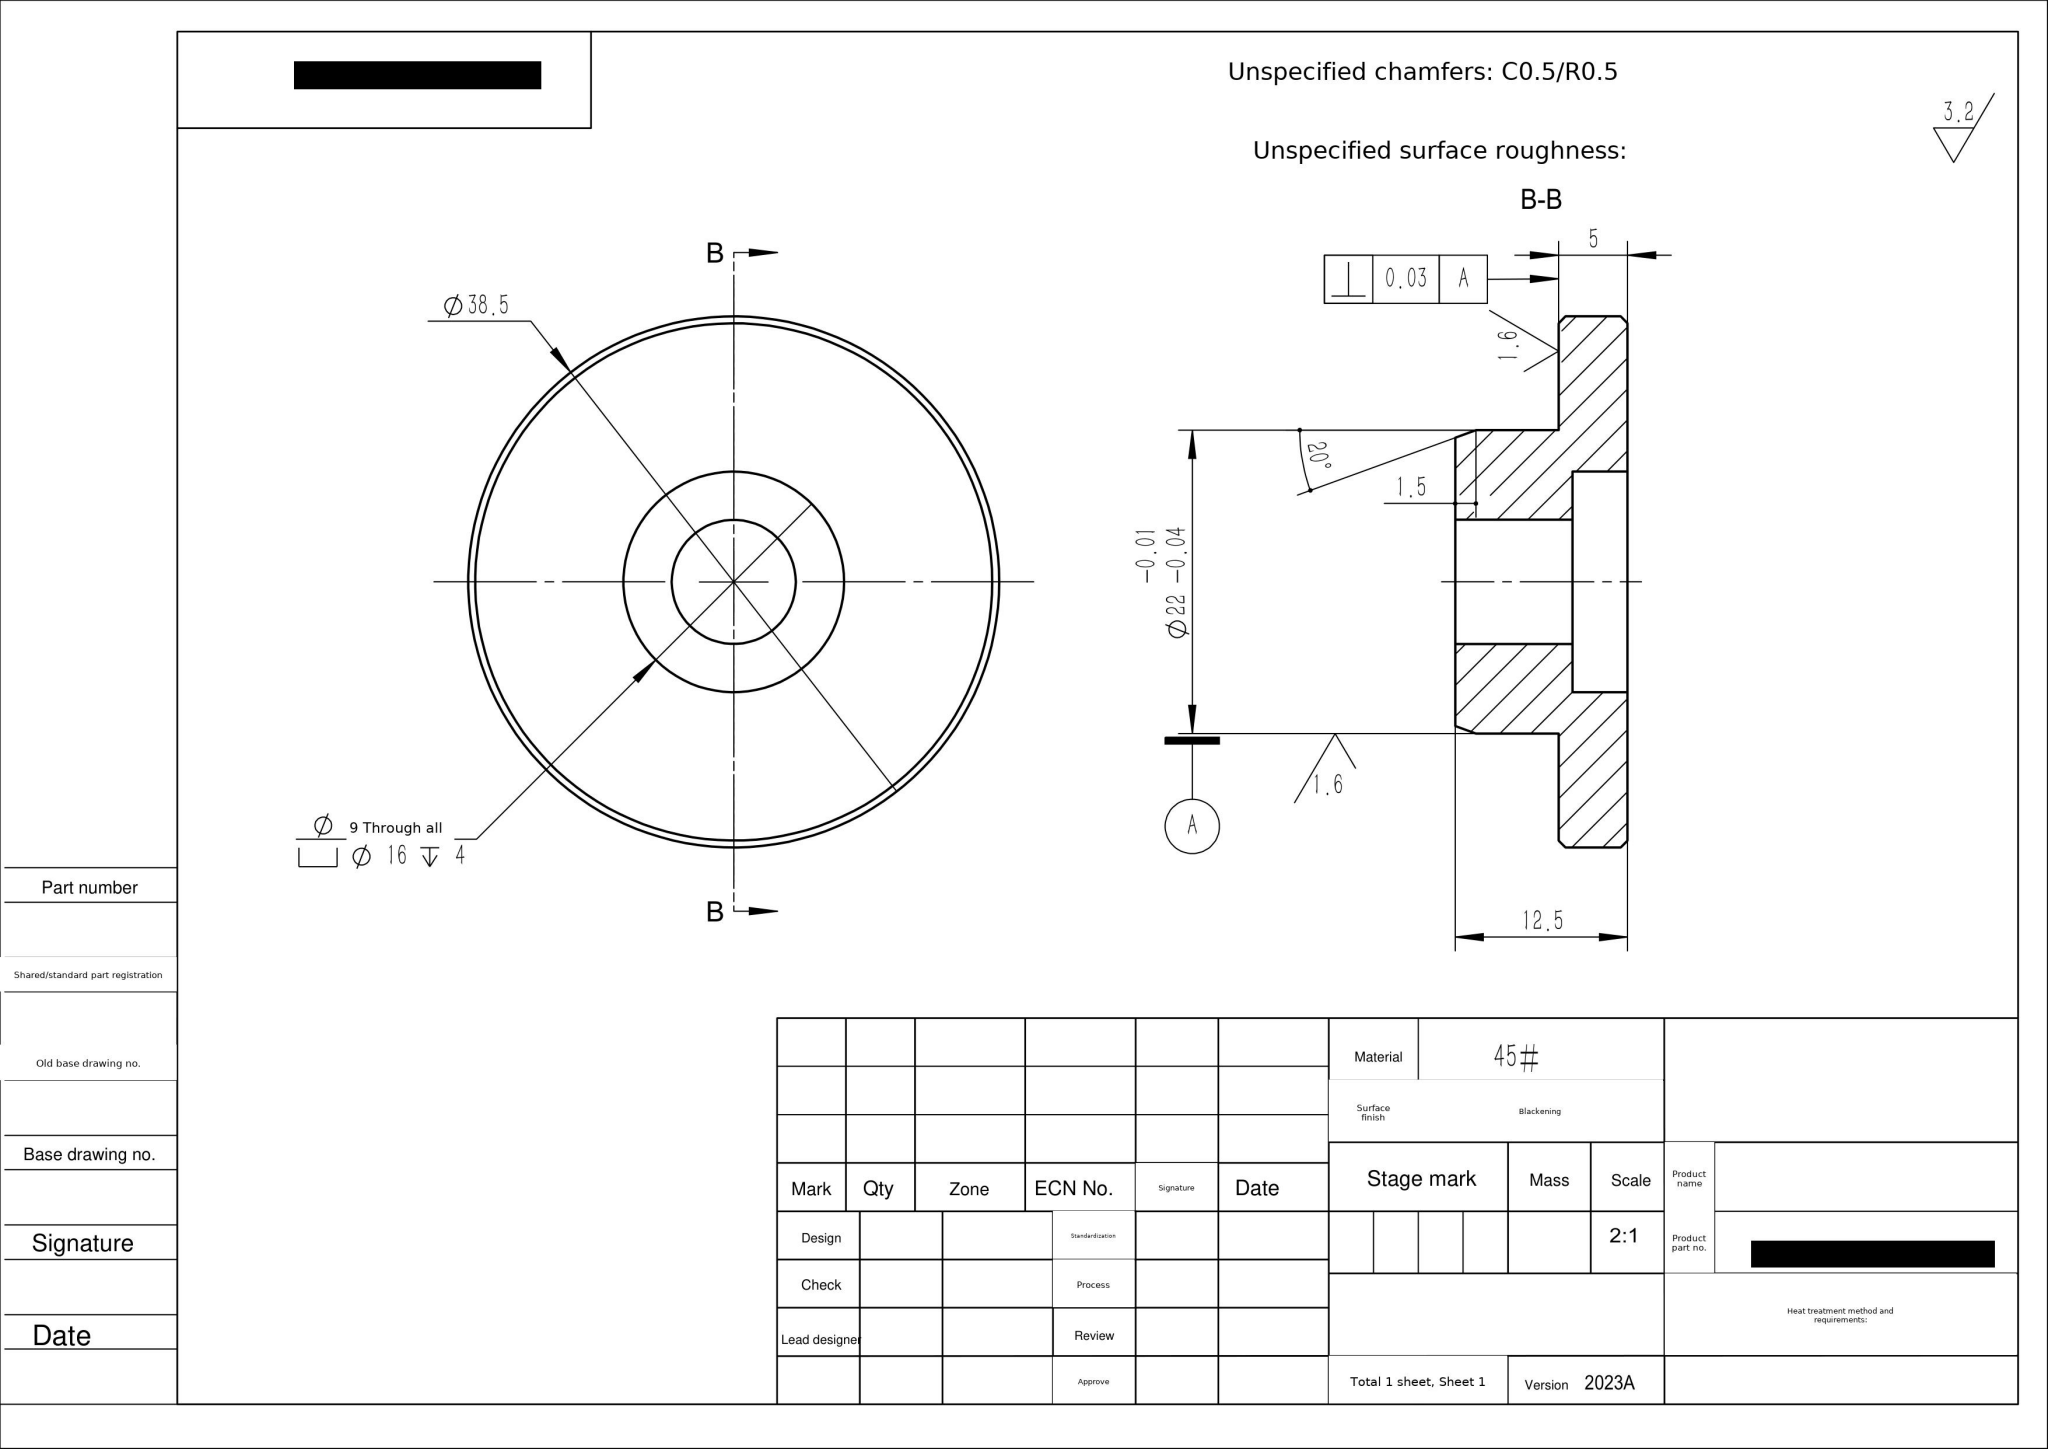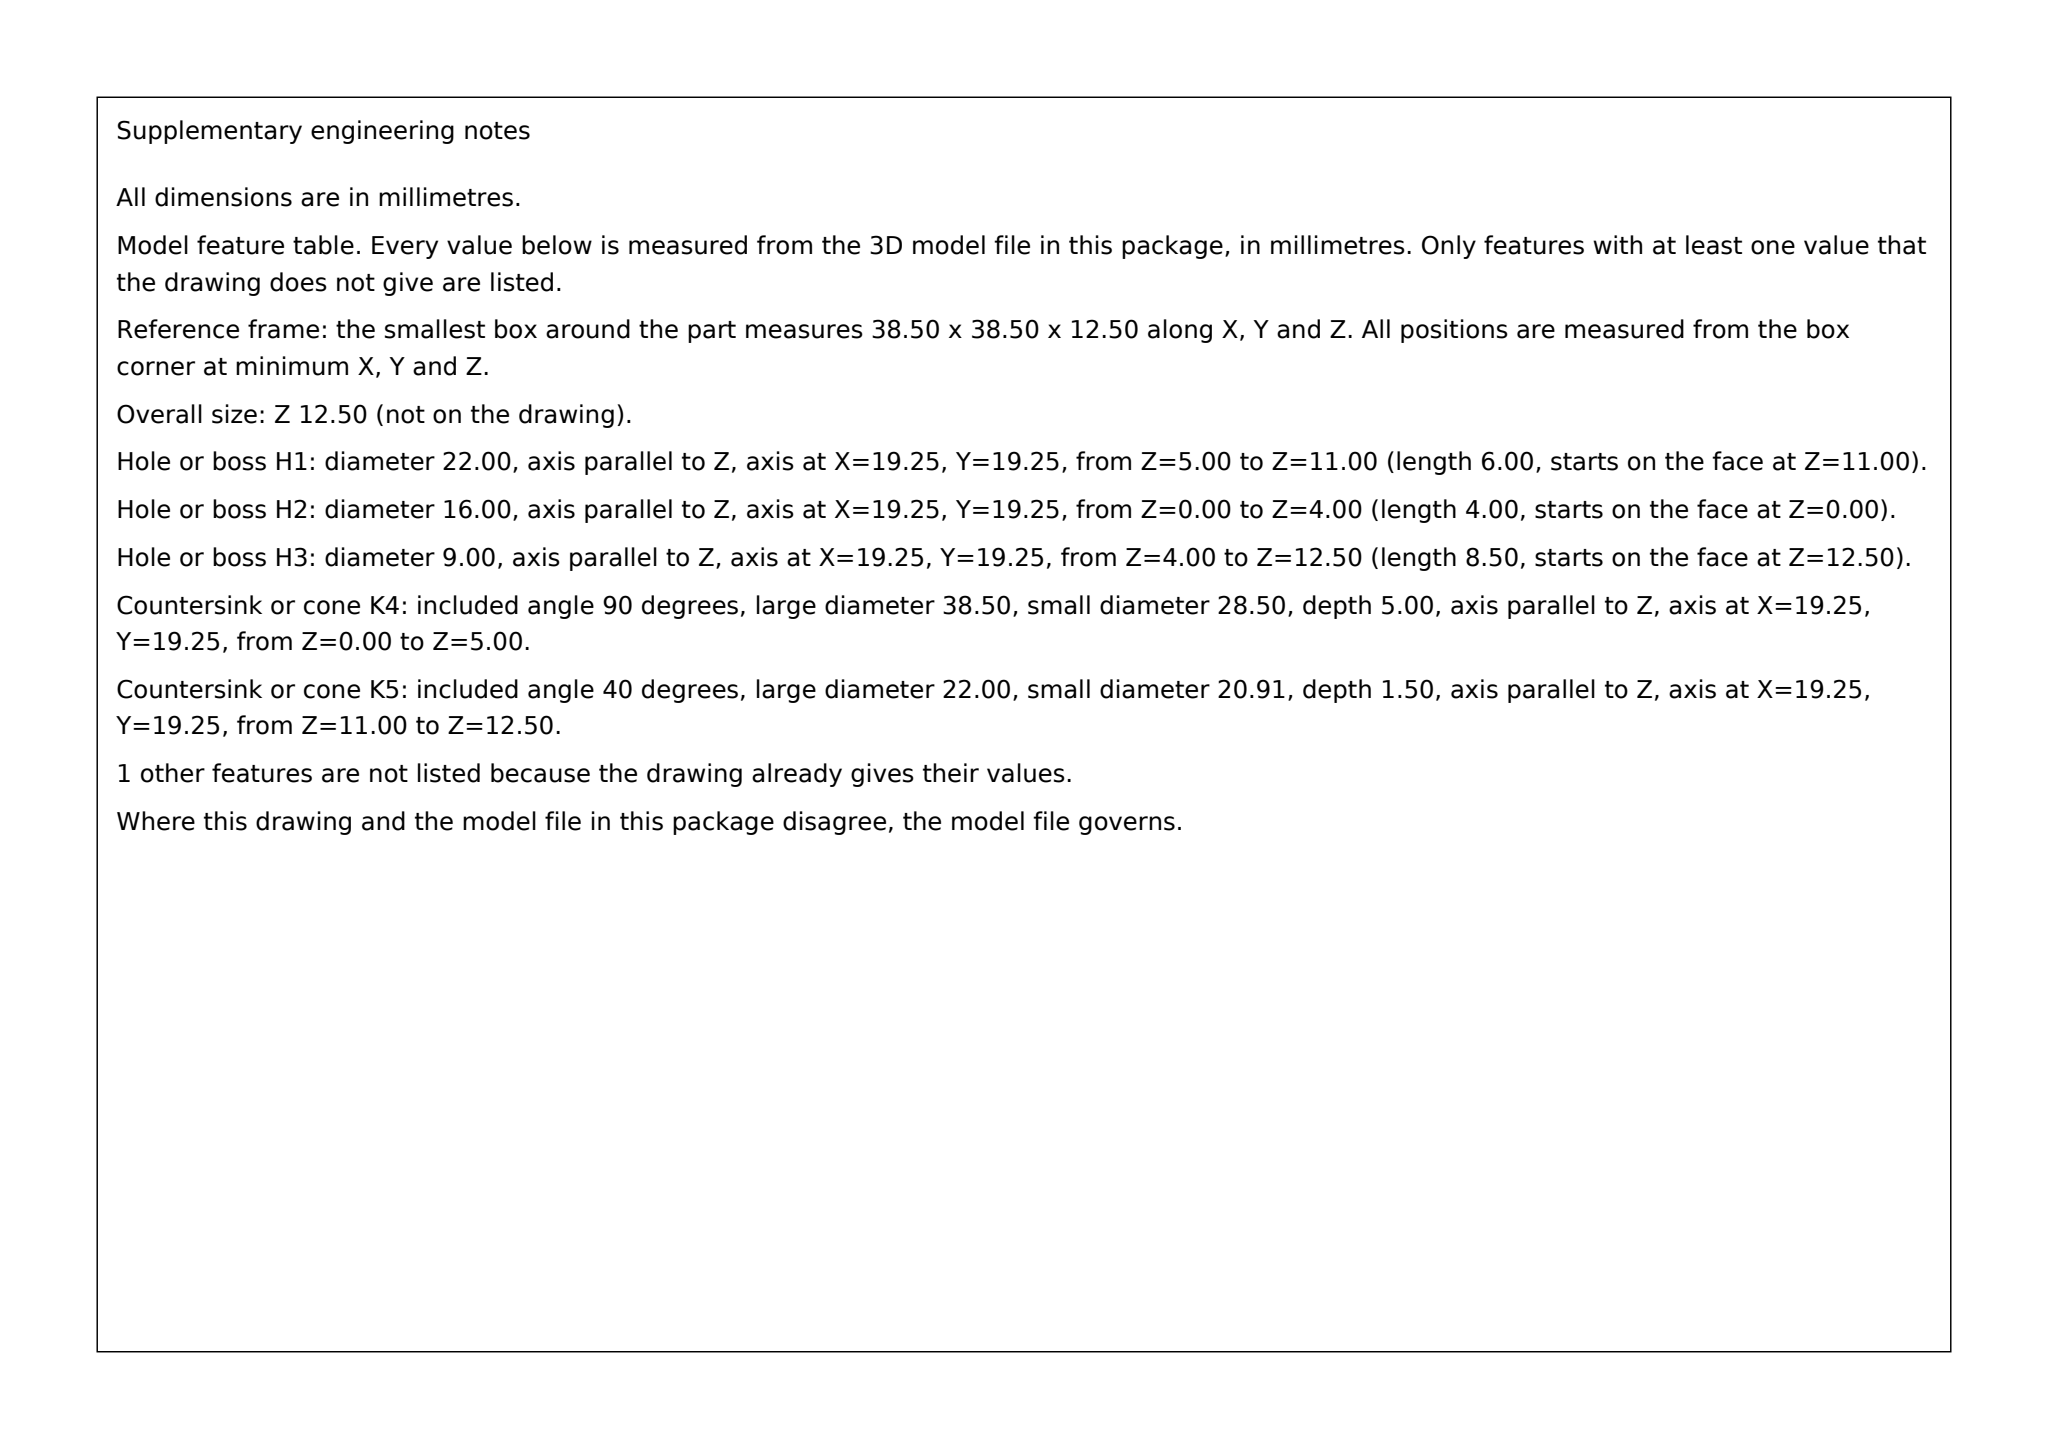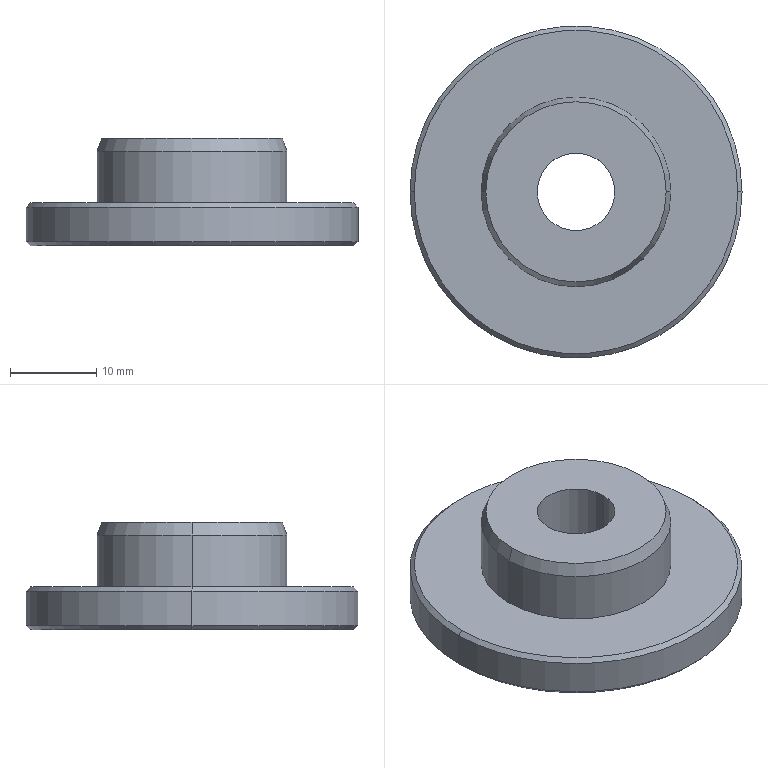Part | SolidWorks | mm | material 45# | 1 solid | 18 faces | box 38.5 x 38.5 x 12.5 mm | volume 7269 mm3 | cylinder 8 | cone 6 | plane 4 | commonest cylinder face diameters 16 x2 9 x2 38.5 x2 22 x2
build123d program:
from build123d import *

# Parameters (mm, degrees)
SKETCH1_R                                            = 11
BOSS_EXTRUDE1_DEPTH                                  = 7.5
SKETCH2_R                                            = 19.25
BOSS_EXTRUDE2_DEPTH                                  = 5
CHAMFER1_SIZE                                        = 1.5
CHAMFER1_SIZE2                                       = 0.546
CHAMFER2_SIZE                                        = 0.5
HOLE_SIZE_ACCORDING_TO_TYPE_1_OF_HEXAGON_D           = 9
HOLE_SIZE_ACCORDING_TO_TYPE_1_OF_HEXAGON_CBORE_D     = 16
HOLE_SIZE_ACCORDING_TO_TYPE_1_OF_HEXAGON_CBORE_DEPTH = 4


with BuildPart() as part:
    # Sketch1 → Boss-Extrude1 (new body)
    with BuildSketch(Plane.XY):
        Circle(SKETCH1_R)
    extrude(amount=BOSS_EXTRUDE1_DEPTH)

    # Sketch2 → Boss-Extrude2 (add)
    with BuildSketch(Plane(origin=(0, 0, 0), x_dir=(-1, 0, 0), z_dir=(0, 0, -1))):
        Circle(SKETCH2_R)
    extrude(amount=BOSS_EXTRUDE2_DEPTH)

    # Chamfer1
    chamfer1_edges = [part.edges().sort_by_distance(p)[0] for p in [
        (-11, 0, 7.5),
    ]]
    chamfer1_side = [part.faces().sort_by_distance(p)[0] for p in [
        (-11, 0, 3.75),
    ]]
    chamfer(chamfer1_edges, length=CHAMFER1_SIZE, length2=CHAMFER1_SIZE2, reference=chamfer1_side[0])

    # Chamfer2
    chamfer2_edges = [part.edges().sort_by_distance(p)[0] for p in [
        (19.25, 0, 0),
        (19.25, 0, -5),
    ]]
    chamfer(chamfer2_edges, length=CHAMFER2_SIZE)

    # Hole Size_According to_Type 1 of Hexagon (through all)
    with Locations(Plane(origin=(0, 0, -5), x_dir=(-1, 0, 0), z_dir=(0, 0, -1))):
        with Locations((0, 0)):
            CounterBoreHole(HOLE_SIZE_ACCORDING_TO_TYPE_1_OF_HEXAGON_D / 2, HOLE_SIZE_ACCORDING_TO_TYPE_1_OF_HEXAGON_CBORE_D / 2, HOLE_SIZE_ACCORDING_TO_TYPE_1_OF_HEXAGON_CBORE_DEPTH)


solid = part.part
STEP:
#1=CARTESIAN_POINT('',(8.,0.,-1.));
#2=VERTEX_POINT('',#1);
#3=CARTESIAN_POINT('',(-8.,0.,-1.));
#4=VERTEX_POINT('',#3);
#5=CARTESIAN_POINT('',(0.,0.,-1.));
#6=DIRECTION('',(0.,0.,-1.));
#7=DIRECTION('',(-1.,0.,0.));
#8=AXIS2_PLACEMENT_3D('',#5,#6,#7);
#9=CIRCLE('',#8,8.);
#10=EDGE_CURVE('',#2,#4,#9,.T.);
#11=ORIENTED_EDGE('',*,*,#10,.F.);
#12=CARTESIAN_POINT('',(8.,0.,-5.));
#13=VERTEX_POINT('',#12);
#14=CARTESIAN_POINT('',(8.,0.,-5.));
#15=DIRECTION('',(0.,0.,-1.));
#16=VECTOR('',#15,1000.);
#17=LINE('',#14,#16);
#18=EDGE_CURVE('',#2,#13,#17,.T.);
#19=ORIENTED_EDGE('',*,*,#18,.T.);
#20=CARTESIAN_POINT('',(-8.,0.,-5.));
#21=VERTEX_POINT('',#20);
#22=CARTESIAN_POINT('',(0.,0.,-5.));
#23=DIRECTION('',(0.,0.,-1.));
#24=DIRECTION('',(-1.,0.,0.));
#25=AXIS2_PLACEMENT_3D('',#22,#23,#24);
#26=CIRCLE('',#25,8.);
#27=EDGE_CURVE('',#13,#21,#26,.T.);
#28=ORIENTED_EDGE('',*,*,#27,.T.);
#29=CARTESIAN_POINT('',(-8.,0.,-5.));
#30=DIRECTION('',(0.,0.,-1.));
#31=VECTOR('',#30,1000.);
#32=LINE('',#29,#31);
#33=EDGE_CURVE('',#4,#21,#32,.T.);
#34=ORIENTED_EDGE('',*,*,#33,.F.);
#35=EDGE_LOOP('',(#11,#19,#28,#34));
#36=FACE_OUTER_BOUND('',#35,.T.);
#37=CARTESIAN_POINT('',(0.,0.,-5.));
#38=DIRECTION('',(0.,0.,-1.));
#39=DIRECTION('',(-1.,0.,0.));
#40=AXIS2_PLACEMENT_3D('',#37,#38,#39);
#41=CYLINDRICAL_SURFACE('',#40,8.);
#42=ADVANCED_FACE('',(#36),#41,.F.);
#43=CARTESIAN_POINT('',(4.5,0.,7.5));
#44=VERTEX_POINT('',#43);
#45=CARTESIAN_POINT('',(-4.5,0.,7.5));
#46=VERTEX_POINT('',#45);
#47=CARTESIAN_POINT('',(0.,0.,7.5));
#48=DIRECTION('',(0.,0.,-1.));
#49=DIRECTION('',(-1.,0.,0.));
#50=AXIS2_PLACEMENT_3D('',#47,#48,#49);
#51=CIRCLE('',#50,4.5);
#52=EDGE_CURVE('',#44,#46,#51,.T.);
#53=ORIENTED_EDGE('',*,*,#52,.F.);
#54=CARTESIAN_POINT('',(4.5,0.,-1.));
#55=VERTEX_POINT('',#54);
#56=CARTESIAN_POINT('',(4.5,0.,-5.));
#57=DIRECTION('',(0.,0.,-1.));
#58=VECTOR('',#57,1000.);
#59=LINE('',#56,#58);
#60=EDGE_CURVE('',#44,#55,#59,.T.);
#61=ORIENTED_EDGE('',*,*,#60,.T.);
#62=CARTESIAN_POINT('',(-4.5,0.,-1.));
#63=VERTEX_POINT('',#62);
#64=CARTESIAN_POINT('',(0.,0.,-1.));
#65=DIRECTION('',(0.,0.,-1.));
#66=DIRECTION('',(-1.,0.,0.));
#67=AXIS2_PLACEMENT_3D('',#64,#65,#66);
#68=CIRCLE('',#67,4.5);
#69=EDGE_CURVE('',#55,#63,#68,.T.);
#70=ORIENTED_EDGE('',*,*,#69,.T.);
#71=CARTESIAN_POINT('',(-4.5,0.,-5.));
#72=DIRECTION('',(0.,0.,-1.));
#73=VECTOR('',#72,1000.);
#74=LINE('',#71,#73);
#75=EDGE_CURVE('',#46,#63,#74,.T.);
#76=ORIENTED_EDGE('',*,*,#75,.F.);
#77=EDGE_LOOP('',(#53,#61,#70,#76));
#78=FACE_OUTER_BOUND('',#77,.T.);
#79=CARTESIAN_POINT('',(0.,0.,-5.));
#80=DIRECTION('',(0.,0.,-1.));
#81=DIRECTION('',(-1.,0.,0.));
#82=AXIS2_PLACEMENT_3D('',#79,#80,#81);
#83=CYLINDRICAL_SURFACE('',#82,4.5);
#84=ADVANCED_FACE('',(#78),#83,.F.);
#85=CARTESIAN_POINT('',(-18.75,0.,-5.));
#86=VERTEX_POINT('',#85);
#87=CARTESIAN_POINT('',(18.75,0.,-5.));
#88=VERTEX_POINT('',#87);
#89=CARTESIAN_POINT('',(0.,0.,-5.));
#90=DIRECTION('',(0.,0.,-1.));
#91=DIRECTION('',(-1.,0.,0.));
#92=AXIS2_PLACEMENT_3D('',#89,#90,#91);
#93=CIRCLE('',#92,18.75);
#94=EDGE_CURVE('',#86,#88,#93,.T.);
#95=ORIENTED_EDGE('',*,*,#94,.F.);
#96=CARTESIAN_POINT('',(-19.25,0.,-4.5));
#97=VERTEX_POINT('',#96);
#98=CARTESIAN_POINT('',(-18.75,0.,-5.));
#99=DIRECTION('',(-0.7071,0.,0.7071));
#100=VECTOR('',#99,1000.);
#101=LINE('',#98,#100);
#102=EDGE_CURVE('',#86,#97,#101,.T.);
#103=ORIENTED_EDGE('',*,*,#102,.T.);
#104=CARTESIAN_POINT('',(19.25,0.,-4.5));
#105=VERTEX_POINT('',#104);
#106=CARTESIAN_POINT('',(0.,0.,-4.5));
#107=DIRECTION('',(0.,0.,1.));
#108=DIRECTION('',(-1.,0.,0.));
#109=AXIS2_PLACEMENT_3D('',#106,#107,#108);
#110=CIRCLE('',#109,19.25);
#111=EDGE_CURVE('',#105,#97,#110,.T.);
#112=ORIENTED_EDGE('',*,*,#111,.F.);
#113=CARTESIAN_POINT('',(18.75,0.,-5.));
#114=DIRECTION('',(0.7071,0.,0.7071));
#115=VECTOR('',#114,1000.);
#116=LINE('',#113,#115);
#117=EDGE_CURVE('',#88,#105,#116,.T.);
#118=ORIENTED_EDGE('',*,*,#117,.F.);
#119=EDGE_LOOP('',(#95,#103,#112,#118));
#120=FACE_OUTER_BOUND('',#119,.T.);
#121=CARTESIAN_POINT('',(0.,0.,-5.));
#122=DIRECTION('',(0.,0.,1.));
#123=DIRECTION('',(1.,0.,0.));
#124=AXIS2_PLACEMENT_3D('',#121,#122,#123);
#125=CONICAL_SURFACE('',#124,18.75,0.7854);
#126=ADVANCED_FACE('',(#120),#125,.T.);
#127=CARTESIAN_POINT('',(18.75,0.,0.));
#128=VERTEX_POINT('',#127);
#129=CARTESIAN_POINT('',(-18.75,0.,0.));
#130=VERTEX_POINT('',#129);
#131=CARTESIAN_POINT('',(0.,0.,0.));
#132=DIRECTION('',(0.,0.,1.));
#133=DIRECTION('',(-1.,0.,0.));
#134=AXIS2_PLACEMENT_3D('',#131,#132,#133);
#135=CIRCLE('',#134,18.75);
#136=EDGE_CURVE('',#128,#130,#135,.T.);
#137=ORIENTED_EDGE('',*,*,#136,.F.);
#138=CARTESIAN_POINT('',(19.25,0.,-0.5));
#139=VERTEX_POINT('',#138);
#140=CARTESIAN_POINT('',(19.25,0.,-0.5));
#141=DIRECTION('',(0.7071,0.,-0.7071));
#142=VECTOR('',#141,1000.);
#143=LINE('',#140,#142);
#144=EDGE_CURVE('',#128,#139,#143,.T.);
#145=ORIENTED_EDGE('',*,*,#144,.T.);
#146=CARTESIAN_POINT('',(-19.25,0.,-0.5));
#147=VERTEX_POINT('',#146);
#148=CARTESIAN_POINT('',(0.,0.,-0.5));
#149=DIRECTION('',(0.,0.,-1.));
#150=DIRECTION('',(-1.,0.,0.));
#151=AXIS2_PLACEMENT_3D('',#148,#149,#150);
#152=CIRCLE('',#151,19.25);
#153=EDGE_CURVE('',#147,#139,#152,.T.);
#154=ORIENTED_EDGE('',*,*,#153,.F.);
#155=CARTESIAN_POINT('',(-19.25,0.,-0.5));
#156=DIRECTION('',(-0.7071,0.,-0.7071));
#157=VECTOR('',#156,1000.);
#158=LINE('',#155,#157);
#159=EDGE_CURVE('',#130,#147,#158,.T.);
#160=ORIENTED_EDGE('',*,*,#159,.F.);
#161=EDGE_LOOP('',(#137,#145,#154,#160));
#162=FACE_OUTER_BOUND('',#161,.T.);
#163=CARTESIAN_POINT('',(0.,0.,-0.5));
#164=DIRECTION('',(0.,0.,-1.));
#165=DIRECTION('',(-1.,0.,0.));
#166=AXIS2_PLACEMENT_3D('',#163,#164,#165);
#167=CONICAL_SURFACE('',#166,19.25,0.7854);
#168=ADVANCED_FACE('',(#162),#167,.T.);
#169=CARTESIAN_POINT('',(10.454,0.,7.5));
#170=VERTEX_POINT('',#169);
#171=CARTESIAN_POINT('',(-10.454,0.,7.5));
#172=VERTEX_POINT('',#171);
#173=CARTESIAN_POINT('',(0.,0.,7.5));
#174=DIRECTION('',(0.,0.,1.));
#175=DIRECTION('',(1.,0.,0.));
#176=AXIS2_PLACEMENT_3D('',#173,#174,#175);
#177=CIRCLE('',#176,10.454);
#178=EDGE_CURVE('',#170,#172,#177,.T.);
#179=ORIENTED_EDGE('',*,*,#178,.F.);
#180=CARTESIAN_POINT('',(11.,0.,6.));
#181=VERTEX_POINT('',#180);
#182=CARTESIAN_POINT('',(10.454,0.,7.5));
#183=DIRECTION('',(0.342,0.,-0.9397));
#184=VECTOR('',#183,1000.);
#185=LINE('',#182,#184);
#186=EDGE_CURVE('',#170,#181,#185,.T.);
#187=ORIENTED_EDGE('',*,*,#186,.T.);
#188=CARTESIAN_POINT('',(-11.,0.,6.));
#189=VERTEX_POINT('',#188);
#190=CARTESIAN_POINT('',(0.,0.,6.));
#191=DIRECTION('',(0.,0.,-1.));
#192=DIRECTION('',(1.,0.,0.));
#193=AXIS2_PLACEMENT_3D('',#190,#191,#192);
#194=CIRCLE('',#193,11.);
#195=EDGE_CURVE('',#189,#181,#194,.T.);
#196=ORIENTED_EDGE('',*,*,#195,.F.);
#197=CARTESIAN_POINT('',(-10.454,0.,7.5));
#198=DIRECTION('',(-0.342,0.,-0.9397));
#199=VECTOR('',#198,1000.);
#200=LINE('',#197,#199);
#201=EDGE_CURVE('',#172,#189,#200,.T.);
#202=ORIENTED_EDGE('',*,*,#201,.F.);
#203=EDGE_LOOP('',(#179,#187,#196,#202));
#204=FACE_OUTER_BOUND('',#203,.T.);
#205=CARTESIAN_POINT('',(0.,0.,7.5));
#206=DIRECTION('',(0.,0.,-1.));
#207=DIRECTION('',(-1.,0.,0.));
#208=AXIS2_PLACEMENT_3D('',#205,#206,#207);
#209=CONICAL_SURFACE('',#208,10.454,0.3491);
#210=ADVANCED_FACE('',(#204),#209,.T.);
#211=ORIENTED_EDGE('',*,*,#111,.T.);
#212=CARTESIAN_POINT('',(-19.25,0.,-5.));
#213=DIRECTION('',(0.,0.,1.));
#214=VECTOR('',#213,1000.);
#215=LINE('',#212,#214);
#216=EDGE_CURVE('',#97,#147,#215,.T.);
#217=ORIENTED_EDGE('',*,*,#216,.T.);
#218=ORIENTED_EDGE('',*,*,#153,.T.);
#219=CARTESIAN_POINT('',(19.25,0.,-5.));
#220=DIRECTION('',(0.,0.,1.));
#221=VECTOR('',#220,1000.);
#222=LINE('',#219,#221);
#223=EDGE_CURVE('',#105,#139,#222,.T.);
#224=ORIENTED_EDGE('',*,*,#223,.F.);
#225=EDGE_LOOP('',(#211,#217,#218,#224));
#226=FACE_OUTER_BOUND('',#225,.T.);
#227=CARTESIAN_POINT('',(0.,0.,-5.));
#228=DIRECTION('',(0.,0.,1.));
#229=DIRECTION('',(1.,0.,0.));
#230=AXIS2_PLACEMENT_3D('',#227,#228,#229);
#231=CYLINDRICAL_SURFACE('',#230,19.25);
#232=ADVANCED_FACE('',(#226),#231,.T.);
#233=ORIENTED_EDGE('',*,*,#195,.T.);
#234=CARTESIAN_POINT('',(11.,0.,0.));
#235=VERTEX_POINT('',#234);
#236=CARTESIAN_POINT('',(11.,0.,7.5));
#237=DIRECTION('',(0.,0.,-1.));
#238=VECTOR('',#237,1000.);
#239=LINE('',#236,#238);
#240=EDGE_CURVE('',#181,#235,#239,.T.);
#241=ORIENTED_EDGE('',*,*,#240,.T.);
#242=CARTESIAN_POINT('',(-11.,0.,0.));
#243=VERTEX_POINT('',#242);
#244=CARTESIAN_POINT('',(0.,0.,0.));
#245=DIRECTION('',(0.,0.,1.));
#246=DIRECTION('',(1.,0.,0.));
#247=AXIS2_PLACEMENT_3D('',#244,#245,#246);
#248=CIRCLE('',#247,11.);
#249=EDGE_CURVE('',#235,#243,#248,.T.);
#250=ORIENTED_EDGE('',*,*,#249,.T.);
#251=CARTESIAN_POINT('',(-11.,0.,7.5));
#252=DIRECTION('',(0.,0.,-1.));
#253=VECTOR('',#252,1000.);
#254=LINE('',#251,#253);
#255=EDGE_CURVE('',#189,#243,#254,.T.);
#256=ORIENTED_EDGE('',*,*,#255,.F.);
#257=EDGE_LOOP('',(#233,#241,#250,#256));
#258=FACE_OUTER_BOUND('',#257,.T.);
#259=CARTESIAN_POINT('',(0.,0.,7.5));
#260=DIRECTION('',(0.,0.,-1.));
#261=DIRECTION('',(-1.,0.,0.));
#262=AXIS2_PLACEMENT_3D('',#259,#260,#261);
#263=CYLINDRICAL_SURFACE('',#262,11.);
#264=ADVANCED_FACE('',(#258),#263,.T.);
#265=ORIENTED_EDGE('',*,*,#240,.F.);
#266=CARTESIAN_POINT('',(0.,0.,6.));
#267=DIRECTION('',(0.,0.,-1.));
#268=DIRECTION('',(1.,0.,0.));
#269=AXIS2_PLACEMENT_3D('',#266,#267,#268);
#270=CIRCLE('',#269,11.);
#271=EDGE_CURVE('',#181,#189,#270,.T.);
#272=ORIENTED_EDGE('',*,*,#271,.T.);
#273=ORIENTED_EDGE('',*,*,#255,.T.);
#274=CARTESIAN_POINT('',(0.,0.,0.));
#275=DIRECTION('',(0.,0.,1.));
#276=DIRECTION('',(1.,0.,0.));
#277=AXIS2_PLACEMENT_3D('',#274,#275,#276);
#278=CIRCLE('',#277,11.);
#279=EDGE_CURVE('',#243,#235,#278,.T.);
#280=ORIENTED_EDGE('',*,*,#279,.T.);
#281=EDGE_LOOP('',(#265,#272,#273,#280));
#282=FACE_OUTER_BOUND('',#281,.T.);
#283=CARTESIAN_POINT('',(0.,0.,7.5));
#284=DIRECTION('',(0.,0.,-1.));
#285=DIRECTION('',(-1.,0.,0.));
#286=AXIS2_PLACEMENT_3D('',#283,#284,#285);
#287=CYLINDRICAL_SURFACE('',#286,11.);
#288=ADVANCED_FACE('',(#282),#287,.T.);
#289=CARTESIAN_POINT('',(0.,0.,7.5));
#290=DIRECTION('',(0.,0.,-1.));
#291=DIRECTION('',(-1.,0.,0.));
#292=AXIS2_PLACEMENT_3D('',#289,#290,#291);
#293=CIRCLE('',#292,4.5);
#294=EDGE_CURVE('',#46,#44,#293,.T.);
#295=ORIENTED_EDGE('',*,*,#294,.T.);
#296=ORIENTED_EDGE('',*,*,#52,.T.);
#297=EDGE_LOOP('',(#295,#296));
#298=FACE_BOUND('',#297,.T.);
#299=CARTESIAN_POINT('',(0.,0.,7.5));
#300=DIRECTION('',(0.,0.,1.));
#301=DIRECTION('',(1.,0.,0.));
#302=AXIS2_PLACEMENT_3D('',#299,#300,#301);
#303=CIRCLE('',#302,10.454);
#304=EDGE_CURVE('',#172,#170,#303,.T.);
#305=ORIENTED_EDGE('',*,*,#304,.T.);
#306=ORIENTED_EDGE('',*,*,#178,.T.);
#307=EDGE_LOOP('',(#305,#306));
#308=FACE_OUTER_BOUND('',#307,.T.);
#309=CARTESIAN_POINT('',(0.,0.,7.5));
#310=DIRECTION('',(0.,0.,1.));
#311=DIRECTION('',(1.,0.,0.));
#312=AXIS2_PLACEMENT_3D('',#309,#310,#311);
#313=PLANE('',#312);
#314=ADVANCED_FACE('',(#298,#308),#313,.T.);
#315=ORIENTED_EDGE('',*,*,#216,.F.);
#316=CARTESIAN_POINT('',(0.,0.,-4.5));
#317=DIRECTION('',(0.,0.,1.));
#318=DIRECTION('',(-1.,0.,0.));
#319=AXIS2_PLACEMENT_3D('',#316,#317,#318);
#320=CIRCLE('',#319,19.25);
#321=EDGE_CURVE('',#97,#105,#320,.T.);
#322=ORIENTED_EDGE('',*,*,#321,.T.);
#323=ORIENTED_EDGE('',*,*,#223,.T.);
#324=CARTESIAN_POINT('',(0.,0.,-0.5));
#325=DIRECTION('',(0.,0.,-1.));
#326=DIRECTION('',(-1.,0.,0.));
#327=AXIS2_PLACEMENT_3D('',#324,#325,#326);
#328=CIRCLE('',#327,19.25);
#329=EDGE_CURVE('',#139,#147,#328,.T.);
#330=ORIENTED_EDGE('',*,*,#329,.T.);
#331=EDGE_LOOP('',(#315,#322,#323,#330));
#332=FACE_OUTER_BOUND('',#331,.T.);
#333=CARTESIAN_POINT('',(0.,0.,-5.));
#334=DIRECTION('',(0.,0.,1.));
#335=DIRECTION('',(1.,0.,0.));
#336=AXIS2_PLACEMENT_3D('',#333,#334,#335);
#337=CYLINDRICAL_SURFACE('',#336,19.25);
#338=ADVANCED_FACE('',(#332),#337,.T.);
#339=CARTESIAN_POINT('',(0.,0.,-5.));
#340=DIRECTION('',(0.,0.,-1.));
#341=DIRECTION('',(-1.,0.,0.));
#342=AXIS2_PLACEMENT_3D('',#339,#340,#341);
#343=CIRCLE('',#342,8.);
#344=EDGE_CURVE('',#21,#13,#343,.T.);
#345=ORIENTED_EDGE('',*,*,#344,.F.);
#346=ORIENTED_EDGE('',*,*,#27,.F.);
#347=EDGE_LOOP('',(#345,#346));
#348=FACE_BOUND('',#347,.T.);
#349=CARTESIAN_POINT('',(0.,0.,-5.));
#350=DIRECTION('',(0.,0.,-1.));
#351=DIRECTION('',(-1.,0.,0.));
#352=AXIS2_PLACEMENT_3D('',#349,#350,#351);
#353=CIRCLE('',#352,18.75);
#354=EDGE_CURVE('',#88,#86,#353,.T.);
#355=ORIENTED_EDGE('',*,*,#354,.T.);
#356=ORIENTED_EDGE('',*,*,#94,.T.);
#357=EDGE_LOOP('',(#355,#356));
#358=FACE_OUTER_BOUND('',#357,.T.);
#359=CARTESIAN_POINT('',(0.,0.,-5.));
#360=DIRECTION('',(0.,0.,-1.));
#361=DIRECTION('',(-1.,0.,0.));
#362=AXIS2_PLACEMENT_3D('',#359,#360,#361);
#363=PLANE('',#362);
#364=ADVANCED_FACE('',(#348,#358),#363,.T.);
#365=CARTESIAN_POINT('',(0.,0.,0.));
#366=DIRECTION('',(0.,0.,1.));
#367=DIRECTION('',(-1.,0.,0.));
#368=AXIS2_PLACEMENT_3D('',#365,#366,#367);
#369=CIRCLE('',#368,18.75);
#370=EDGE_CURVE('',#130,#128,#369,.T.);
#371=ORIENTED_EDGE('',*,*,#370,.T.);
#372=ORIENTED_EDGE('',*,*,#136,.T.);
#373=EDGE_LOOP('',(#371,#372));
#374=FACE_OUTER_BOUND('',#373,.T.);
#375=ORIENTED_EDGE('',*,*,#279,.F.);
#376=ORIENTED_EDGE('',*,*,#249,.F.);
#377=EDGE_LOOP('',(#375,#376));
#378=FACE_BOUND('',#377,.T.);
#379=CARTESIAN_POINT('',(0.,0.,0.));
#380=DIRECTION('',(0.,0.,-1.));
#381=DIRECTION('',(-1.,0.,0.));
#382=AXIS2_PLACEMENT_3D('',#379,#380,#381);
#383=PLANE('',#382);
#384=ADVANCED_FACE('',(#374,#378),#383,.F.);
#385=ORIENTED_EDGE('',*,*,#186,.F.);
#386=ORIENTED_EDGE('',*,*,#304,.F.);
#387=ORIENTED_EDGE('',*,*,#201,.T.);
#388=ORIENTED_EDGE('',*,*,#271,.F.);
#389=EDGE_LOOP('',(#385,#386,#387,#388));
#390=FACE_OUTER_BOUND('',#389,.T.);
#391=CARTESIAN_POINT('',(0.,0.,7.5));
#392=DIRECTION('',(0.,0.,-1.));
#393=DIRECTION('',(-1.,0.,0.));
#394=AXIS2_PLACEMENT_3D('',#391,#392,#393);
#395=CONICAL_SURFACE('',#394,10.454,0.3491);
#396=ADVANCED_FACE('',(#390),#395,.T.);
#397=ORIENTED_EDGE('',*,*,#144,.F.);
#398=ORIENTED_EDGE('',*,*,#370,.F.);
#399=ORIENTED_EDGE('',*,*,#159,.T.);
#400=ORIENTED_EDGE('',*,*,#329,.F.);
#401=EDGE_LOOP('',(#397,#398,#399,#400));
#402=FACE_OUTER_BOUND('',#401,.T.);
#403=CARTESIAN_POINT('',(0.,0.,-0.5));
#404=DIRECTION('',(0.,0.,-1.));
#405=DIRECTION('',(-1.,0.,0.));
#406=AXIS2_PLACEMENT_3D('',#403,#404,#405);
#407=CONICAL_SURFACE('',#406,19.25,0.7854);
#408=ADVANCED_FACE('',(#402),#407,.T.);
#409=ORIENTED_EDGE('',*,*,#102,.F.);
#410=ORIENTED_EDGE('',*,*,#354,.F.);
#411=ORIENTED_EDGE('',*,*,#117,.T.);
#412=ORIENTED_EDGE('',*,*,#321,.F.);
#413=EDGE_LOOP('',(#409,#410,#411,#412));
#414=FACE_OUTER_BOUND('',#413,.T.);
#415=CARTESIAN_POINT('',(0.,0.,-5.));
#416=DIRECTION('',(0.,0.,1.));
#417=DIRECTION('',(1.,0.,0.));
#418=AXIS2_PLACEMENT_3D('',#415,#416,#417);
#419=CONICAL_SURFACE('',#418,18.75,0.7854);
#420=ADVANCED_FACE('',(#414),#419,.T.);
#421=ORIENTED_EDGE('',*,*,#60,.F.);
#422=ORIENTED_EDGE('',*,*,#294,.F.);
#423=ORIENTED_EDGE('',*,*,#75,.T.);
#424=CARTESIAN_POINT('',(0.,0.,-1.));
#425=DIRECTION('',(0.,0.,-1.));
#426=DIRECTION('',(-1.,0.,0.));
#427=AXIS2_PLACEMENT_3D('',#424,#425,#426);
#428=CIRCLE('',#427,4.5);
#429=EDGE_CURVE('',#63,#55,#428,.T.);
#430=ORIENTED_EDGE('',*,*,#429,.T.);
#431=EDGE_LOOP('',(#421,#422,#423,#430));
#432=FACE_OUTER_BOUND('',#431,.T.);
#433=CARTESIAN_POINT('',(0.,0.,-5.));
#434=DIRECTION('',(0.,0.,-1.));
#435=DIRECTION('',(-1.,0.,0.));
#436=AXIS2_PLACEMENT_3D('',#433,#434,#435);
#437=CYLINDRICAL_SURFACE('',#436,4.5);
#438=ADVANCED_FACE('',(#432),#437,.F.);
#439=ORIENTED_EDGE('',*,*,#429,.F.);
#440=ORIENTED_EDGE('',*,*,#69,.F.);
#441=EDGE_LOOP('',(#439,#440));
#442=FACE_BOUND('',#441,.T.);
#443=CARTESIAN_POINT('',(0.,0.,-1.));
#444=DIRECTION('',(0.,0.,-1.));
#445=DIRECTION('',(-1.,0.,0.));
#446=AXIS2_PLACEMENT_3D('',#443,#444,#445);
#447=CIRCLE('',#446,8.);
#448=EDGE_CURVE('',#4,#2,#447,.T.);
#449=ORIENTED_EDGE('',*,*,#448,.T.);
#450=ORIENTED_EDGE('',*,*,#10,.T.);
#451=EDGE_LOOP('',(#449,#450));
#452=FACE_OUTER_BOUND('',#451,.T.);
#453=CARTESIAN_POINT('',(4.5,0.,-1.));
#454=DIRECTION('',(0.,0.,1.));
#455=DIRECTION('',(1.,0.,0.));
#456=AXIS2_PLACEMENT_3D('',#453,#454,#455);
#457=PLANE('',#456);
#458=ADVANCED_FACE('',(#442,#452),#457,.F.);
#459=ORIENTED_EDGE('',*,*,#18,.F.);
#460=ORIENTED_EDGE('',*,*,#448,.F.);
#461=ORIENTED_EDGE('',*,*,#33,.T.);
#462=ORIENTED_EDGE('',*,*,#344,.T.);
#463=EDGE_LOOP('',(#459,#460,#461,#462));
#464=FACE_OUTER_BOUND('',#463,.T.);
#465=CARTESIAN_POINT('',(0.,0.,-5.));
#466=DIRECTION('',(0.,0.,-1.));
#467=DIRECTION('',(-1.,0.,0.));
#468=AXIS2_PLACEMENT_3D('',#465,#466,#467);
#469=CYLINDRICAL_SURFACE('',#468,8.);
#470=ADVANCED_FACE('',(#464),#469,.F.);
#471=CLOSED_SHELL('',(#42,#84,#126,#168,#210,#232,#264,#288,#314,#338,#364,#384,#396,#408,#420,#438,#458,#470));
#472=MANIFOLD_SOLID_BREP('',#471);
#473=CARTESIAN_POINT('',(0.,0.,0.));
#474=DIRECTION('',(0.,0.,1.));
#475=DIRECTION('',(1.,0.,0.));
#476=AXIS2_PLACEMENT_3D('',#473,#474,#475);
#477=(LENGTH_UNIT()NAMED_UNIT(*)SI_UNIT(.MILLI.,.METRE.));
#478=UNCERTAINTY_MEASURE_WITH_UNIT(LENGTH_MEASURE(0.00001),#477,'','');
#479=(NAMED_UNIT(*)PLANE_ANGLE_UNIT()SI_UNIT($,.RADIAN.));
#480=(NAMED_UNIT(*)SI_UNIT($,.STERADIAN.)SOLID_ANGLE_UNIT());
#481=(GEOMETRIC_REPRESENTATION_CONTEXT(3)GLOBAL_UNCERTAINTY_ASSIGNED_CONTEXT((#478))GLOBAL_UNIT_ASSIGNED_CONTEXT((#477,#479,#480))REPRESENTATION_CONTEXT('',''));
#482=ADVANCED_BREP_SHAPE_REPRESENTATION('',(#472,#476),#481);